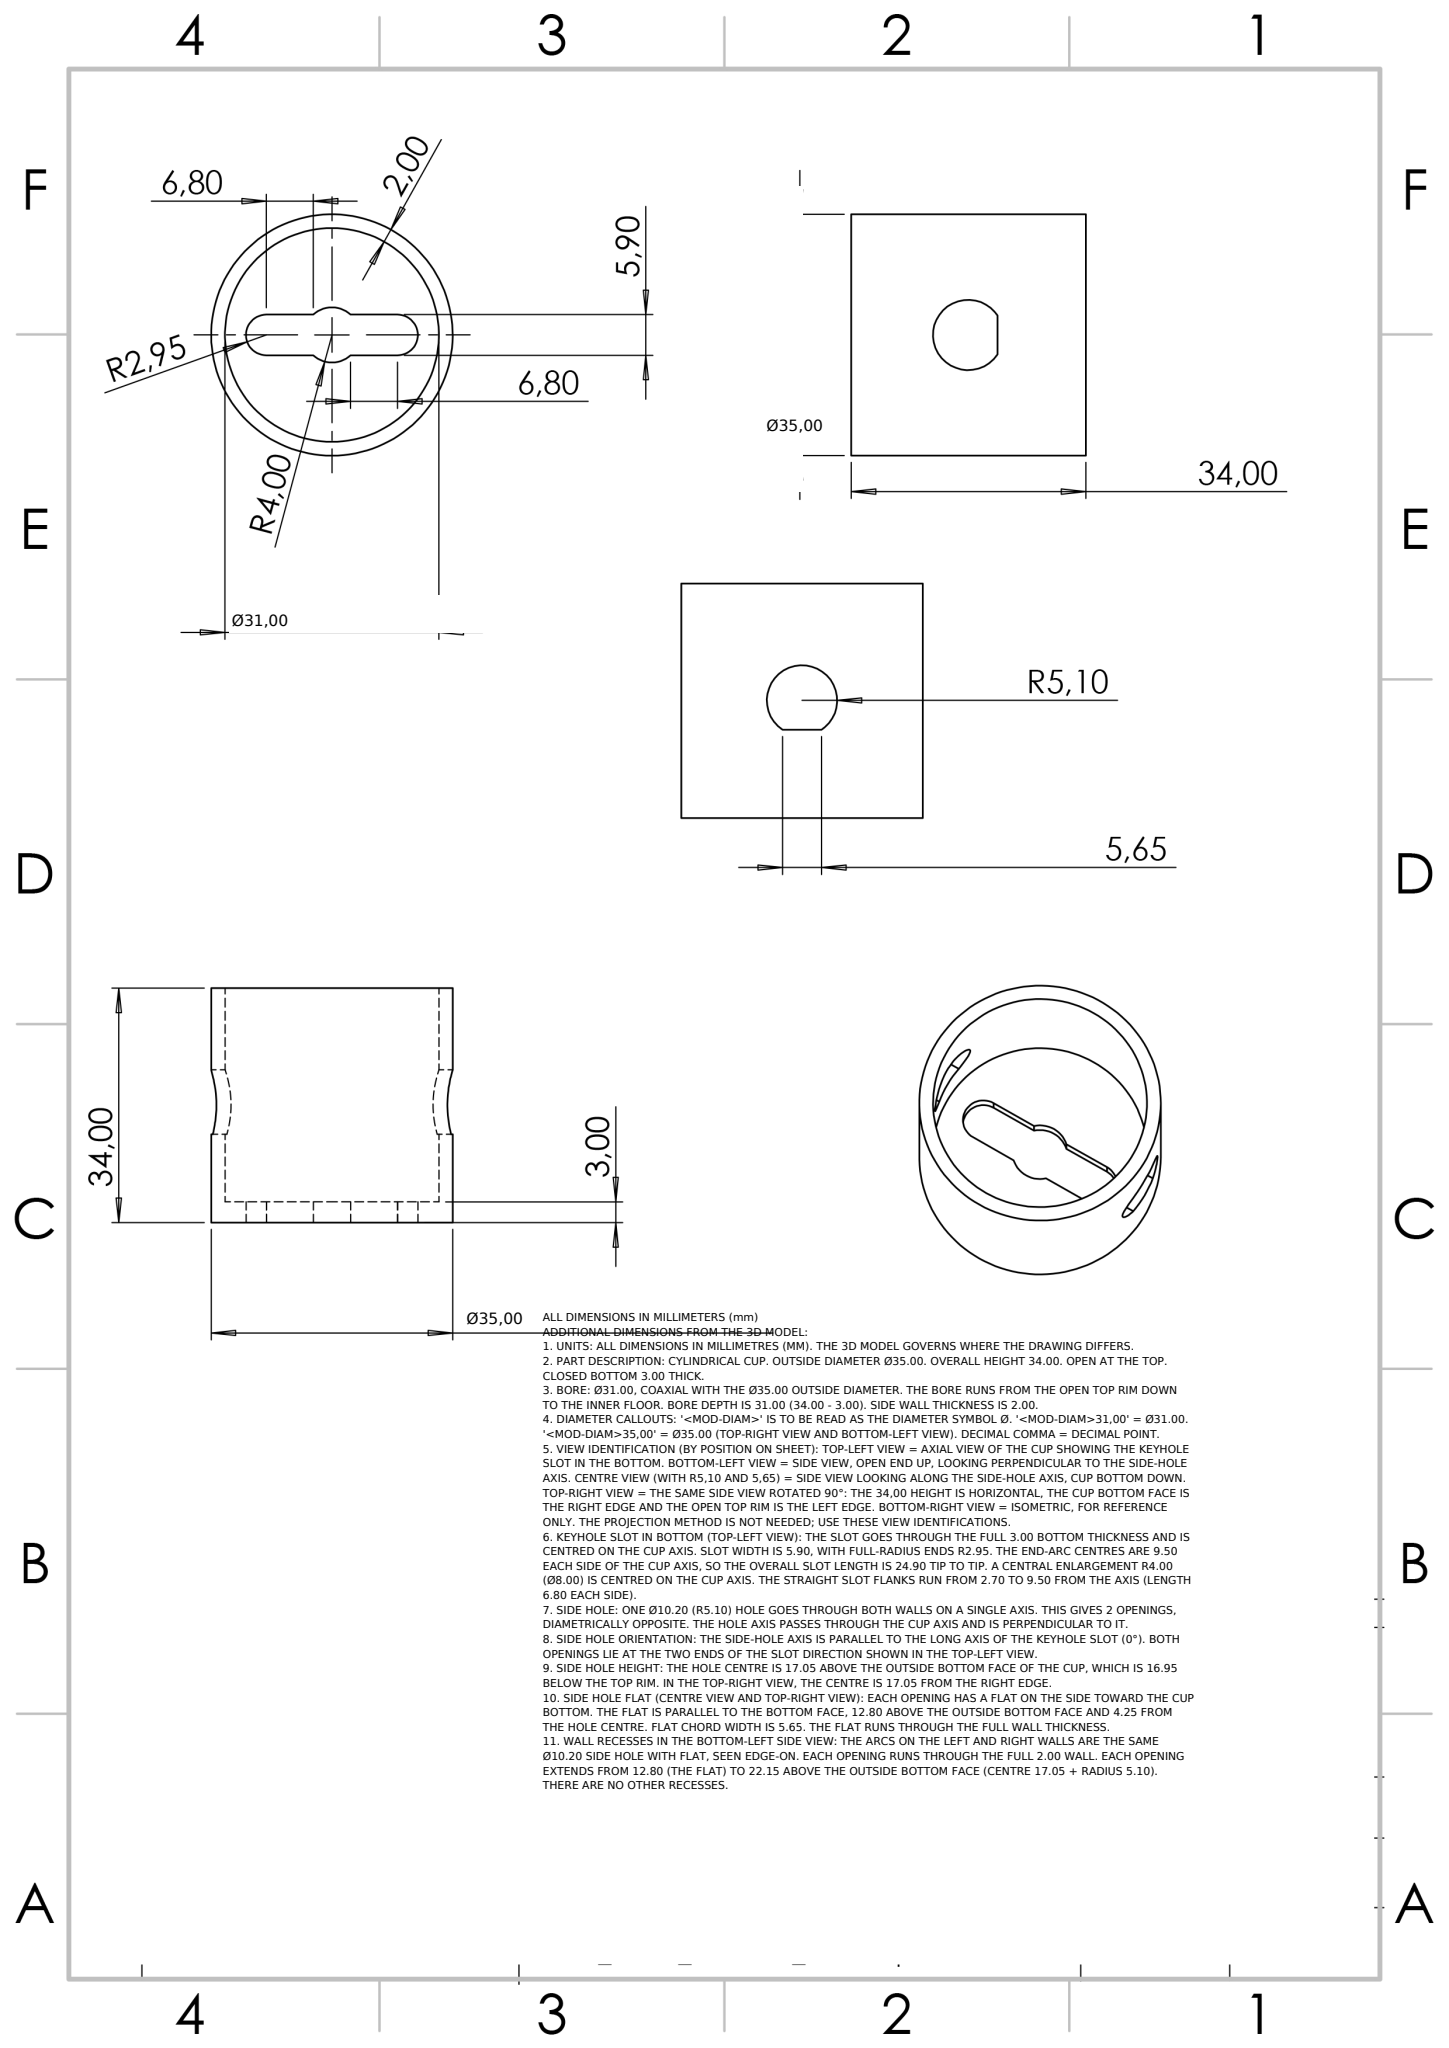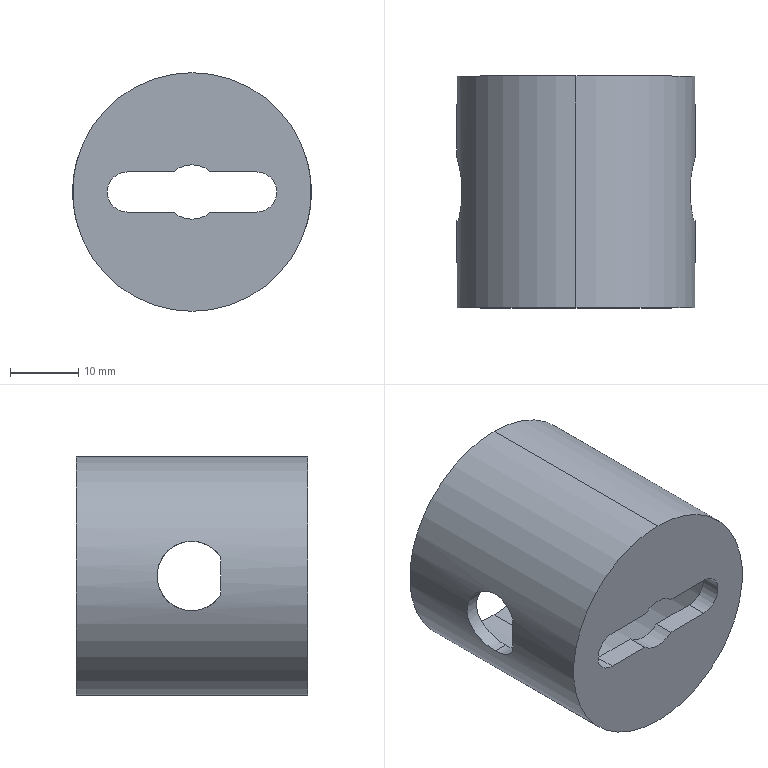Part | NX | mm | 1 solid | 24 faces | box 35 x 34 x 35 mm | volume 8555 mm3 | cylinder 15 | plane 9 | commonest cylinder face diameters 10.2 x6 8 x3 31 x2 35 x2 5.9 x2